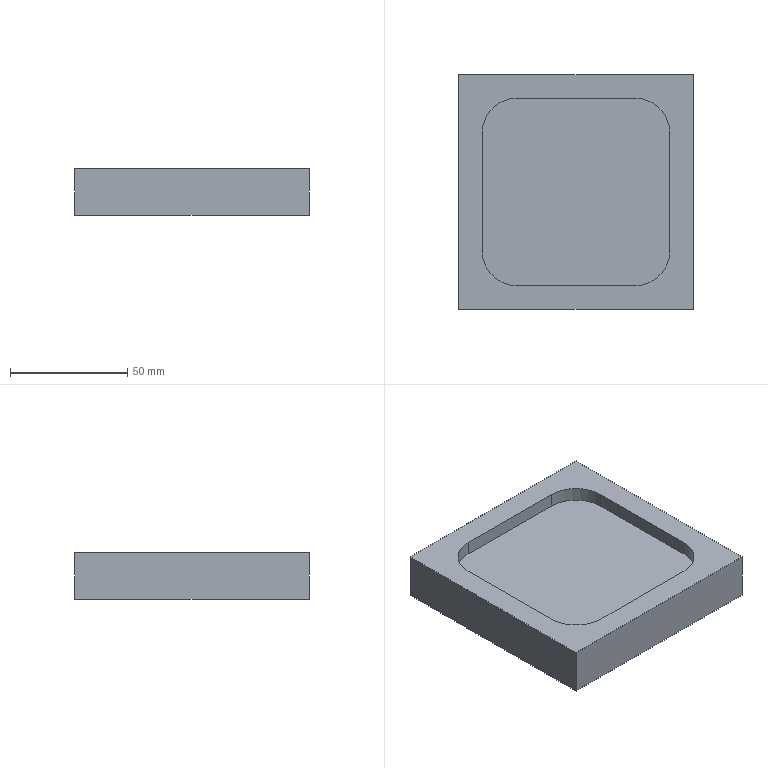CAM job | NX | mm | 3-axis | 1 set-up | 5 operations | part box 100 x 100 x 20
set-up 1
1. Face Milling | Mill Mill5 D12 | FACE_MILLING | path 9522.762 mm | 2.992 min
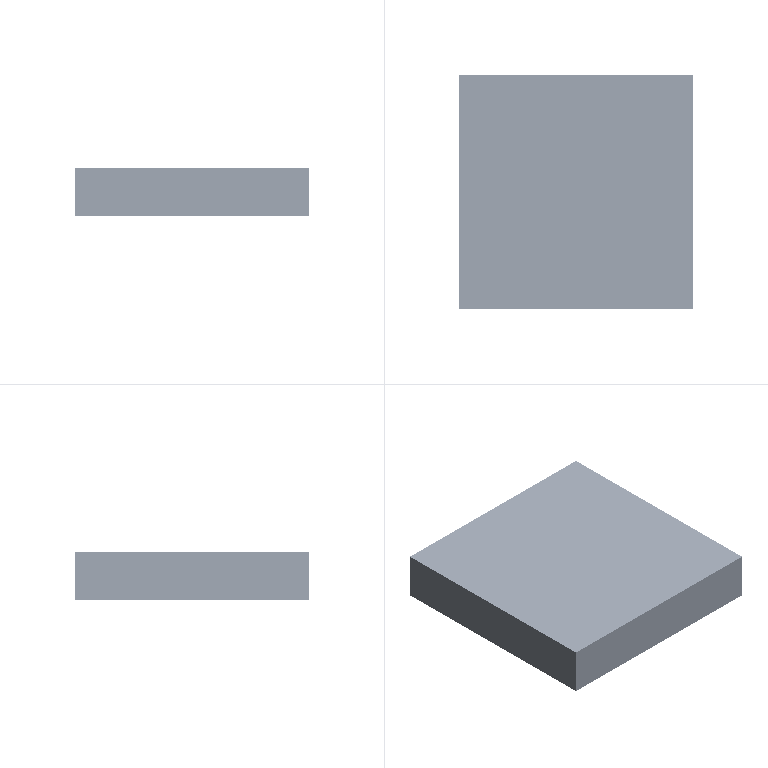2. Cavity Milling | Mill Mill5 D12 | CAVITY_MILL | path 18426.316 mm | 5.77 min
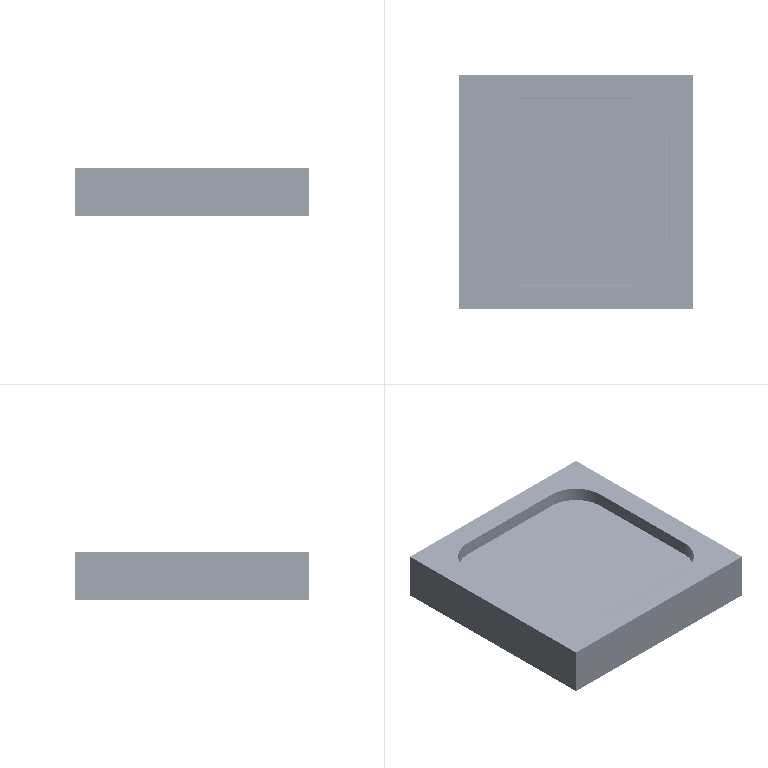3. Face Milling | Mill Mill5 D12 | FACE_MILLING_COPY | path 1510.769 mm | 2.433 min
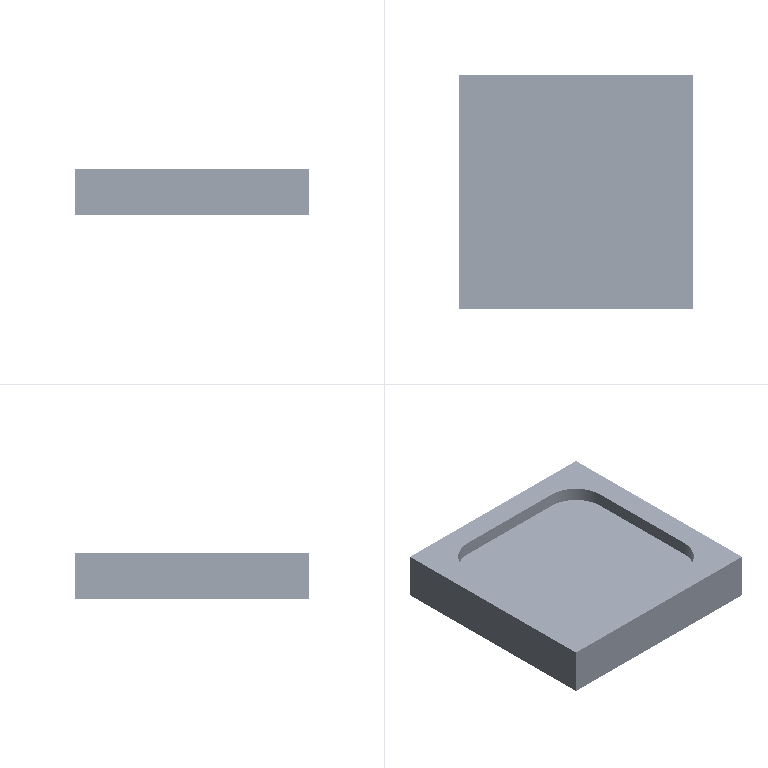4. Cavity Milling | Mill Mill5 D12 | CAVITY_MILL_COPY | path 1020.393 mm | 1.611 min
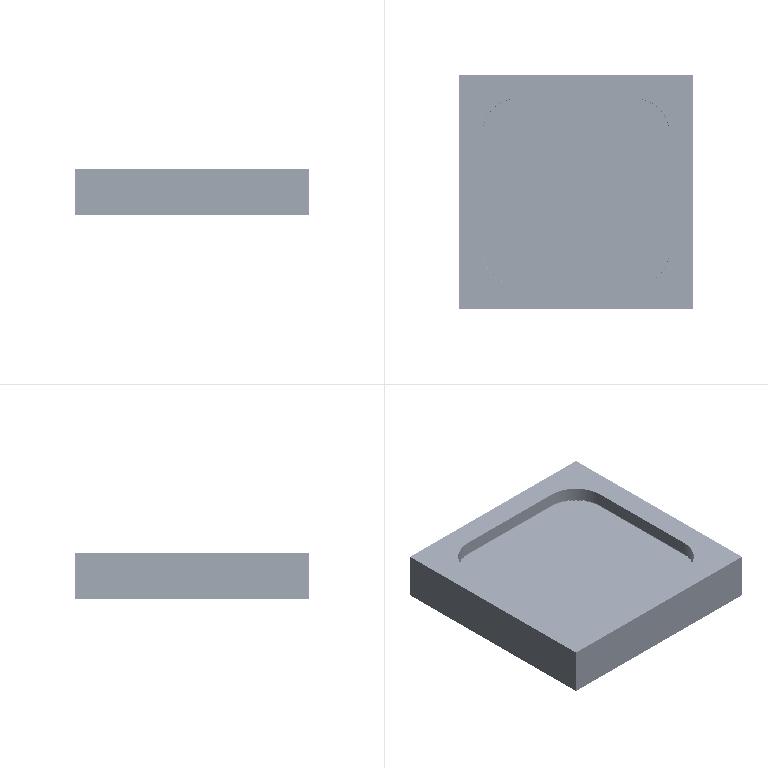5. Cavity Milling | Mill Mill5 D12 | CAVITY_MILL_COPY_COPY | path 351.648 mm | 0.4827 min